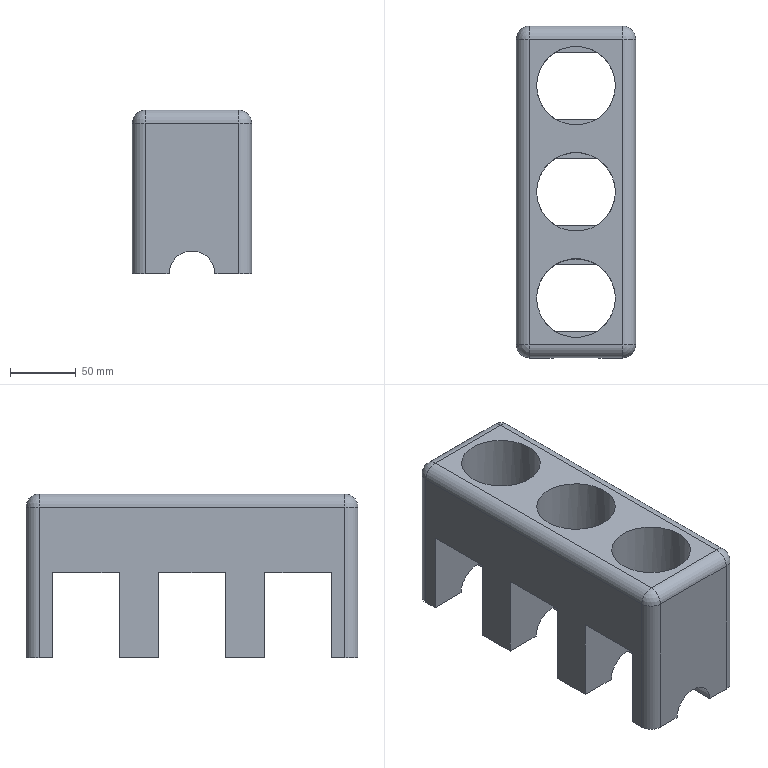Component | NX | HOUSING | 1 solid | 50 faces | volume 1376964 mm3 | plane 31 | cylinder 15 | sphere 4 | commonest cylinder face diameters 20 x8 35 x4 60.1 x3